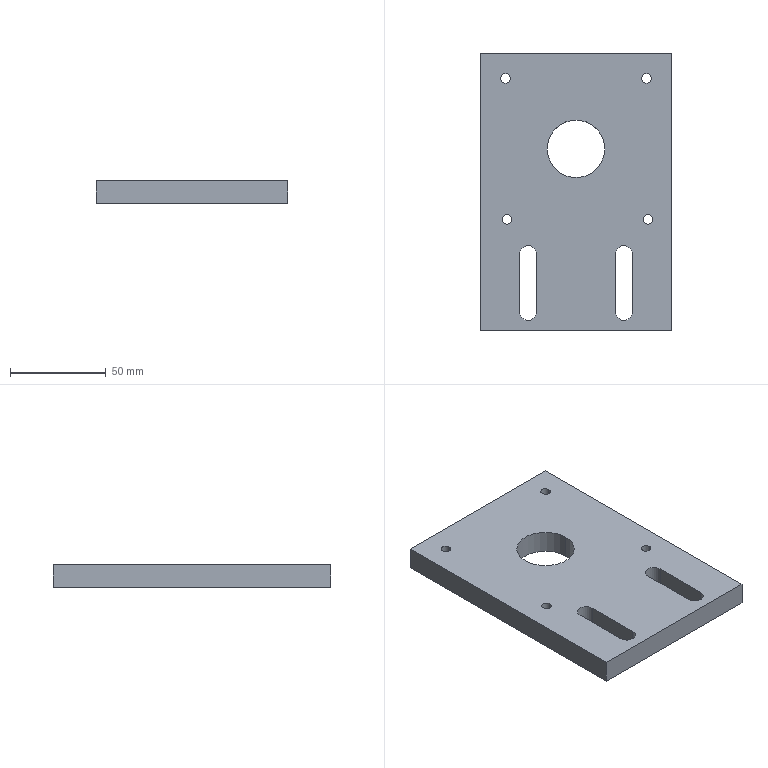Component | SolidWorks | MotorMount-2 | 1 solid | 24 faces | box 100 x 145 x 12 mm | volume 156568 mm3 | cylinder 14 | plane 10 | commonest cylinder face diameters 5 x8 9 x4 30 x2
build123d program:
from build123d import *

# Parameters (mm, degrees)
SKETCH1_W             = 100
SKETCH1_H             = 145
SKETCH1_R             = 15
EXTRUDE1_DEPTH        = 12
M6_TAPPED_HOLE1_D     = 5
M6_TAPPED_HOLE1_DEPTH = 17
M6_TAPPED_HOLE1_TIP   = 1.502


with BuildPart() as part:
    # Sketch1 → Extrude1 (new body)
    with BuildSketch(Plane.XY):
        with Locations((25.043, -0.7753)):
            Rectangle(SKETCH1_W, SKETCH1_H)
        with Locations((25.043, 21.725)):
            Circle(SKETCH1_R, mode=Mode.SUBTRACT)
        with BuildLine():
            Line((45.543, -33.275), (45.543, -63.275))
            ThreePointArc((45.543, -63.275), (50.043, -67.775), (54.543, -63.275))
            Line((54.543, -63.275), (54.543, -33.275))
            ThreePointArc((54.543, -33.275), (50.043, -28.775), (45.543, -33.275))
        make_face(mode=Mode.SUBTRACT)
        with BuildLine():
            Line((-4.457, -33.275), (-4.457, -63.275))
            ThreePointArc((-4.457, -63.275), (0.04302, -67.775), (4.543, -63.275))
            Line((4.543, -63.275), (4.543, -33.275))
            ThreePointArc((4.543, -33.275), (0.04302, -28.775), (-4.457, -33.275))
        make_face(mode=Mode.SUBTRACT)
    extrude(amount=EXTRUDE1_DEPTH)

    # M6 Tapped Hole1
    with Locations(Plane(origin=(0, 0, 0), x_dir=(-1, 0, 0), z_dir=(0, 0, -1))):
        with Locations((11.707, 58.475), (-61.793, 58.475), (-62.543, -15.021), (10.957, -15.025)):
            Hole(M6_TAPPED_HOLE1_D / 2, depth=M6_TAPPED_HOLE1_DEPTH)
            with Locations((0, 0, -(M6_TAPPED_HOLE1_DEPTH + M6_TAPPED_HOLE1_TIP / 2))):  # 118° drill point
                Cone(0, M6_TAPPED_HOLE1_D / 2, M6_TAPPED_HOLE1_TIP, mode=Mode.SUBTRACT)


solid = part.part

# Placed as in the assembly
solid = solid.moved(Location((-185.987, 672.259, 237.789), (0, 0, 0)))
STEP:
#1=COLOUR_RGB('',0.7922,0.8196,0.9333);
#2=FILL_AREA_STYLE_COLOUR('',#1);
#3=FILL_AREA_STYLE('',(#2));
#4=SURFACE_STYLE_FILL_AREA(#3);
#5=SURFACE_SIDE_STYLE('',(#4));
#6=SURFACE_STYLE_USAGE(.BOTH.,#5);
#7=PRESENTATION_STYLE_ASSIGNMENT((#6));
#8=CARTESIAN_POINT('',(-7.882,28.769,9.834));
#9=VERTEX_POINT('',#8);
#10=CARTESIAN_POINT('',(-7.685,28.769,9.834));
#11=VERTEX_POINT('',#10);
#12=CARTESIAN_POINT('',(-7.783,28.769,9.834));
#13=DIRECTION('',(0.,0.,1.));
#14=DIRECTION('',(1.,0.,0.));
#15=AXIS2_PLACEMENT_3D('',#12,#13,#14);
#16=CIRCLE('',#15,0.09843);
#17=EDGE_CURVE('',#9,#11,#16,.T.);
#18=ORIENTED_EDGE('',*,*,#17,.T.);
#19=CARTESIAN_POINT('',(-7.685,28.769,9.362));
#20=VERTEX_POINT('',#19);
#21=CARTESIAN_POINT('',(-7.685,28.769,9.362));
#22=DIRECTION('',(0.,0.,-1.));
#23=VECTOR('',#22,39.37);
#24=LINE('',#21,#23);
#25=EDGE_CURVE('',#11,#20,#24,.T.);
#26=ORIENTED_EDGE('',*,*,#25,.T.);
#27=CARTESIAN_POINT('',(-7.882,28.769,9.362));
#28=VERTEX_POINT('',#27);
#29=CARTESIAN_POINT('',(-7.783,28.769,9.362));
#30=DIRECTION('',(0.,0.,-1.));
#31=DIRECTION('',(-1.,0.,0.));
#32=AXIS2_PLACEMENT_3D('',#29,#30,#31);
#33=CIRCLE('',#32,0.09843);
#34=EDGE_CURVE('',#20,#28,#33,.T.);
#35=ORIENTED_EDGE('',*,*,#34,.T.);
#36=CARTESIAN_POINT('',(-7.882,28.769,9.362));
#37=DIRECTION('',(0.,0.,-1.));
#38=VECTOR('',#37,39.37);
#39=LINE('',#36,#38);
#40=EDGE_CURVE('',#9,#28,#39,.T.);
#41=ORIENTED_EDGE('',*,*,#40,.F.);
#42=EDGE_LOOP('',(#18,#26,#35,#41));
#43=FACE_OUTER_BOUND('',#42,.T.);
#44=CARTESIAN_POINT('',(-7.783,28.769,9.362));
#45=DIRECTION('',(0.,0.,-1.));
#46=DIRECTION('',(-1.,0.,0.));
#47=AXIS2_PLACEMENT_3D('',#44,#45,#46);
#48=CYLINDRICAL_SURFACE('',#47,0.09843);
#49=ADVANCED_FACE('',(#43),#48,.F.);
#50=CARTESIAN_POINT('',(-4.988,28.769,9.834));
#51=VERTEX_POINT('',#50);
#52=CARTESIAN_POINT('',(-4.791,28.769,9.834));
#53=VERTEX_POINT('',#52);
#54=CARTESIAN_POINT('',(-4.89,28.769,9.834));
#55=DIRECTION('',(0.,0.,1.));
#56=DIRECTION('',(1.,0.,0.));
#57=AXIS2_PLACEMENT_3D('',#54,#55,#56);
#58=CIRCLE('',#57,0.09843);
#59=EDGE_CURVE('',#51,#53,#58,.T.);
#60=ORIENTED_EDGE('',*,*,#59,.T.);
#61=CARTESIAN_POINT('',(-4.791,28.769,9.362));
#62=VERTEX_POINT('',#61);
#63=CARTESIAN_POINT('',(-4.791,28.769,9.362));
#64=DIRECTION('',(0.,0.,-1.));
#65=VECTOR('',#64,39.37);
#66=LINE('',#63,#65);
#67=EDGE_CURVE('',#53,#62,#66,.T.);
#68=ORIENTED_EDGE('',*,*,#67,.T.);
#69=CARTESIAN_POINT('',(-4.988,28.769,9.362));
#70=VERTEX_POINT('',#69);
#71=CARTESIAN_POINT('',(-4.89,28.769,9.362));
#72=DIRECTION('',(0.,0.,-1.));
#73=DIRECTION('',(-1.,0.,0.));
#74=AXIS2_PLACEMENT_3D('',#71,#72,#73);
#75=CIRCLE('',#74,0.09843);
#76=EDGE_CURVE('',#62,#70,#75,.T.);
#77=ORIENTED_EDGE('',*,*,#76,.T.);
#78=CARTESIAN_POINT('',(-4.988,28.769,9.362));
#79=DIRECTION('',(0.,0.,-1.));
#80=VECTOR('',#79,39.37);
#81=LINE('',#78,#80);
#82=EDGE_CURVE('',#51,#70,#81,.T.);
#83=ORIENTED_EDGE('',*,*,#82,.F.);
#84=EDGE_LOOP('',(#60,#68,#77,#83));
#85=FACE_OUTER_BOUND('',#84,.T.);
#86=CARTESIAN_POINT('',(-4.89,28.769,9.362));
#87=DIRECTION('',(0.,0.,-1.));
#88=DIRECTION('',(-1.,0.,0.));
#89=AXIS2_PLACEMENT_3D('',#86,#87,#88);
#90=CYLINDRICAL_SURFACE('',#89,0.09843);
#91=ADVANCED_FACE('',(#85),#90,.F.);
#92=CARTESIAN_POINT('',(-4.958,25.875,9.834));
#93=VERTEX_POINT('',#92);
#94=CARTESIAN_POINT('',(-4.762,25.875,9.834));
#95=VERTEX_POINT('',#94);
#96=CARTESIAN_POINT('',(-4.86,25.875,9.834));
#97=DIRECTION('',(0.,0.,1.));
#98=DIRECTION('',(1.,0.,0.));
#99=AXIS2_PLACEMENT_3D('',#96,#97,#98);
#100=CIRCLE('',#99,0.09843);
#101=EDGE_CURVE('',#93,#95,#100,.T.);
#102=ORIENTED_EDGE('',*,*,#101,.T.);
#103=CARTESIAN_POINT('',(-4.762,25.875,9.362));
#104=VERTEX_POINT('',#103);
#105=CARTESIAN_POINT('',(-4.762,25.875,9.362));
#106=DIRECTION('',(0.,0.,-1.));
#107=VECTOR('',#106,39.37);
#108=LINE('',#105,#107);
#109=EDGE_CURVE('',#95,#104,#108,.T.);
#110=ORIENTED_EDGE('',*,*,#109,.T.);
#111=CARTESIAN_POINT('',(-4.958,25.875,9.362));
#112=VERTEX_POINT('',#111);
#113=CARTESIAN_POINT('',(-4.86,25.875,9.362));
#114=DIRECTION('',(0.,0.,-1.));
#115=DIRECTION('',(-1.,0.,0.));
#116=AXIS2_PLACEMENT_3D('',#113,#114,#115);
#117=CIRCLE('',#116,0.09843);
#118=EDGE_CURVE('',#104,#112,#117,.T.);
#119=ORIENTED_EDGE('',*,*,#118,.T.);
#120=CARTESIAN_POINT('',(-4.958,25.875,9.362));
#121=DIRECTION('',(0.,0.,-1.));
#122=VECTOR('',#121,39.37);
#123=LINE('',#120,#122);
#124=EDGE_CURVE('',#93,#112,#123,.T.);
#125=ORIENTED_EDGE('',*,*,#124,.F.);
#126=EDGE_LOOP('',(#102,#110,#119,#125));
#127=FACE_OUTER_BOUND('',#126,.T.);
#128=CARTESIAN_POINT('',(-4.86,25.875,9.362));
#129=DIRECTION('',(0.,0.,-1.));
#130=DIRECTION('',(-1.,0.,0.));
#131=AXIS2_PLACEMENT_3D('',#128,#129,#130);
#132=CYLINDRICAL_SURFACE('',#131,0.09843);
#133=ADVANCED_FACE('',(#127),#132,.F.);
#134=CARTESIAN_POINT('',(-7.852,25.875,9.834));
#135=VERTEX_POINT('',#134);
#136=CARTESIAN_POINT('',(-7.655,25.875,9.834));
#137=VERTEX_POINT('',#136);
#138=CARTESIAN_POINT('',(-7.754,25.875,9.834));
#139=DIRECTION('',(0.,0.,1.));
#140=DIRECTION('',(1.,0.,0.));
#141=AXIS2_PLACEMENT_3D('',#138,#139,#140);
#142=CIRCLE('',#141,0.09843);
#143=EDGE_CURVE('',#135,#137,#142,.T.);
#144=ORIENTED_EDGE('',*,*,#143,.T.);
#145=CARTESIAN_POINT('',(-7.655,25.875,9.362));
#146=VERTEX_POINT('',#145);
#147=CARTESIAN_POINT('',(-7.655,25.875,9.362));
#148=DIRECTION('',(0.,0.,-1.));
#149=VECTOR('',#148,39.37);
#150=LINE('',#147,#149);
#151=EDGE_CURVE('',#137,#146,#150,.T.);
#152=ORIENTED_EDGE('',*,*,#151,.T.);
#153=CARTESIAN_POINT('',(-7.852,25.875,9.362));
#154=VERTEX_POINT('',#153);
#155=CARTESIAN_POINT('',(-7.754,25.875,9.362));
#156=DIRECTION('',(0.,0.,-1.));
#157=DIRECTION('',(-1.,0.,0.));
#158=AXIS2_PLACEMENT_3D('',#155,#156,#157);
#159=CIRCLE('',#158,0.09843);
#160=EDGE_CURVE('',#146,#154,#159,.T.);
#161=ORIENTED_EDGE('',*,*,#160,.T.);
#162=CARTESIAN_POINT('',(-7.852,25.875,9.362));
#163=DIRECTION('',(0.,0.,-1.));
#164=VECTOR('',#163,39.37);
#165=LINE('',#162,#164);
#166=EDGE_CURVE('',#135,#154,#165,.T.);
#167=ORIENTED_EDGE('',*,*,#166,.F.);
#168=EDGE_LOOP('',(#144,#152,#161,#167));
#169=FACE_OUTER_BOUND('',#168,.T.);
#170=CARTESIAN_POINT('',(-7.754,25.875,9.362));
#171=DIRECTION('',(0.,0.,-1.));
#172=DIRECTION('',(-1.,0.,0.));
#173=AXIS2_PLACEMENT_3D('',#170,#171,#172);
#174=CYLINDRICAL_SURFACE('',#173,0.09843);
#175=ADVANCED_FACE('',(#169),#174,.F.);
#176=CARTESIAN_POINT('',(-6.927,27.322,9.834));
#177=VERTEX_POINT('',#176);
#178=CARTESIAN_POINT('',(-5.746,27.322,9.834));
#179=VERTEX_POINT('',#178);
#180=CARTESIAN_POINT('',(-6.336,27.322,9.834));
#181=DIRECTION('',(0.,0.,1.));
#182=DIRECTION('',(1.,0.,0.));
#183=AXIS2_PLACEMENT_3D('',#180,#181,#182);
#184=CIRCLE('',#183,0.5906);
#185=EDGE_CURVE('',#177,#179,#184,.T.);
#186=ORIENTED_EDGE('',*,*,#185,.T.);
#187=CARTESIAN_POINT('',(-5.746,27.322,9.362));
#188=VERTEX_POINT('',#187);
#189=CARTESIAN_POINT('',(-5.746,27.322,9.834));
#190=DIRECTION('',(0.,0.,-1.));
#191=VECTOR('',#190,39.37);
#192=LINE('',#189,#191);
#193=EDGE_CURVE('',#179,#188,#192,.T.);
#194=ORIENTED_EDGE('',*,*,#193,.T.);
#195=CARTESIAN_POINT('',(-6.927,27.322,9.362));
#196=VERTEX_POINT('',#195);
#197=CARTESIAN_POINT('',(-6.336,27.322,9.362));
#198=DIRECTION('',(0.,0.,1.));
#199=DIRECTION('',(1.,0.,0.));
#200=AXIS2_PLACEMENT_3D('',#197,#198,#199);
#201=CIRCLE('',#200,0.5906);
#202=EDGE_CURVE('',#196,#188,#201,.T.);
#203=ORIENTED_EDGE('',*,*,#202,.F.);
#204=CARTESIAN_POINT('',(-6.927,27.322,9.834));
#205=DIRECTION('',(0.,0.,-1.));
#206=VECTOR('',#205,39.37);
#207=LINE('',#204,#206);
#208=EDGE_CURVE('',#177,#196,#207,.T.);
#209=ORIENTED_EDGE('',*,*,#208,.F.);
#210=EDGE_LOOP('',(#186,#194,#203,#209));
#211=FACE_OUTER_BOUND('',#210,.T.);
#212=CARTESIAN_POINT('',(-6.336,27.322,9.834));
#213=DIRECTION('',(0.,0.,-1.));
#214=DIRECTION('',(-1.,0.,0.));
#215=AXIS2_PLACEMENT_3D('',#212,#213,#214);
#216=CYLINDRICAL_SURFACE('',#215,0.5906);
#217=ADVANCED_FACE('',(#211),#216,.F.);
#218=ORIENTED_EDGE('',*,*,#17,.F.);
#219=CARTESIAN_POINT('',(-7.783,28.769,9.834));
#220=DIRECTION('',(0.,0.,1.));
#221=DIRECTION('',(1.,0.,0.));
#222=AXIS2_PLACEMENT_3D('',#219,#220,#221);
#223=CIRCLE('',#222,0.09843);
#224=EDGE_CURVE('',#11,#9,#223,.T.);
#225=ORIENTED_EDGE('',*,*,#224,.F.);
#226=EDGE_LOOP('',(#218,#225));
#227=FACE_BOUND('',#226,.T.);
#228=ORIENTED_EDGE('',*,*,#59,.F.);
#229=CARTESIAN_POINT('',(-4.89,28.769,9.834));
#230=DIRECTION('',(0.,0.,1.));
#231=DIRECTION('',(1.,0.,0.));
#232=AXIS2_PLACEMENT_3D('',#229,#230,#231);
#233=CIRCLE('',#232,0.09843);
#234=EDGE_CURVE('',#53,#51,#233,.T.);
#235=ORIENTED_EDGE('',*,*,#234,.F.);
#236=EDGE_LOOP('',(#228,#235));
#237=FACE_BOUND('',#236,.T.);
#238=ORIENTED_EDGE('',*,*,#101,.F.);
#239=CARTESIAN_POINT('',(-4.86,25.875,9.834));
#240=DIRECTION('',(0.,0.,1.));
#241=DIRECTION('',(1.,0.,0.));
#242=AXIS2_PLACEMENT_3D('',#239,#240,#241);
#243=CIRCLE('',#242,0.09843);
#244=EDGE_CURVE('',#95,#93,#243,.T.);
#245=ORIENTED_EDGE('',*,*,#244,.F.);
#246=EDGE_LOOP('',(#238,#245));
#247=FACE_BOUND('',#246,.T.);
#248=ORIENTED_EDGE('',*,*,#143,.F.);
#249=CARTESIAN_POINT('',(-7.754,25.875,9.834));
#250=DIRECTION('',(0.,0.,1.));
#251=DIRECTION('',(1.,0.,0.));
#252=AXIS2_PLACEMENT_3D('',#249,#250,#251);
#253=CIRCLE('',#252,0.09843);
#254=EDGE_CURVE('',#137,#135,#253,.T.);
#255=ORIENTED_EDGE('',*,*,#254,.F.);
#256=EDGE_LOOP('',(#248,#255));
#257=FACE_BOUND('',#256,.T.);
#258=CARTESIAN_POINT('',(-8.305,29.291,9.834));
#259=VERTEX_POINT('',#258);
#260=CARTESIAN_POINT('',(-8.305,23.582,9.834));
#261=VERTEX_POINT('',#260);
#262=CARTESIAN_POINT('',(-8.305,29.291,9.834));
#263=DIRECTION('',(0.,-1.,0.));
#264=VECTOR('',#263,39.37);
#265=LINE('',#262,#264);
#266=EDGE_CURVE('',#259,#261,#265,.T.);
#267=ORIENTED_EDGE('',*,*,#266,.T.);
#268=CARTESIAN_POINT('',(-4.368,23.582,9.834));
#269=VERTEX_POINT('',#268);
#270=CARTESIAN_POINT('',(-8.305,23.582,9.834));
#271=DIRECTION('',(1.,0.,0.));
#272=VECTOR('',#271,39.37);
#273=LINE('',#270,#272);
#274=EDGE_CURVE('',#261,#269,#273,.T.);
#275=ORIENTED_EDGE('',*,*,#274,.T.);
#276=CARTESIAN_POINT('',(-4.368,29.291,9.834));
#277=VERTEX_POINT('',#276);
#278=CARTESIAN_POINT('',(-4.368,29.291,9.834));
#279=DIRECTION('',(-0.,1.,0.));
#280=VECTOR('',#279,39.37);
#281=LINE('',#278,#280);
#282=EDGE_CURVE('',#269,#277,#281,.T.);
#283=ORIENTED_EDGE('',*,*,#282,.T.);
#284=CARTESIAN_POINT('',(-8.305,29.291,9.834));
#285=DIRECTION('',(-1.,0.,0.));
#286=VECTOR('',#285,39.37);
#287=LINE('',#284,#286);
#288=EDGE_CURVE('',#277,#259,#287,.T.);
#289=ORIENTED_EDGE('',*,*,#288,.T.);
#290=EDGE_LOOP('',(#267,#275,#283,#289));
#291=FACE_OUTER_BOUND('',#290,.T.);
#292=ORIENTED_EDGE('',*,*,#185,.F.);
#293=CARTESIAN_POINT('',(-6.336,27.322,9.834));
#294=DIRECTION('',(0.,0.,1.));
#295=DIRECTION('',(1.,0.,0.));
#296=AXIS2_PLACEMENT_3D('',#293,#294,#295);
#297=CIRCLE('',#296,0.5906);
#298=EDGE_CURVE('',#179,#177,#297,.T.);
#299=ORIENTED_EDGE('',*,*,#298,.F.);
#300=EDGE_LOOP('',(#292,#299));
#301=FACE_BOUND('',#300,.T.);
#302=CARTESIAN_POINT('',(-7.498,25.157,9.834));
#303=VERTEX_POINT('',#302);
#304=CARTESIAN_POINT('',(-7.498,23.976,9.834));
#305=VERTEX_POINT('',#304);
#306=CARTESIAN_POINT('',(-7.498,25.157,9.834));
#307=DIRECTION('',(0.,-1.,0.));
#308=VECTOR('',#307,39.37);
#309=LINE('',#306,#308);
#310=EDGE_CURVE('',#303,#305,#309,.T.);
#311=ORIENTED_EDGE('',*,*,#310,.F.);
#312=CARTESIAN_POINT('',(-7.143,25.157,9.834));
#313=VERTEX_POINT('',#312);
#314=CARTESIAN_POINT('',(-7.321,25.157,9.834));
#315=DIRECTION('',(0.,0.,1.));
#316=DIRECTION('',(1.,0.,0.));
#317=AXIS2_PLACEMENT_3D('',#314,#315,#316);
#318=CIRCLE('',#317,0.1772);
#319=EDGE_CURVE('',#313,#303,#318,.T.);
#320=ORIENTED_EDGE('',*,*,#319,.F.);
#321=CARTESIAN_POINT('',(-7.143,23.976,9.834));
#322=VERTEX_POINT('',#321);
#323=CARTESIAN_POINT('',(-7.143,25.157,9.834));
#324=DIRECTION('',(-0.,1.,0.));
#325=VECTOR('',#324,39.37);
#326=LINE('',#323,#325);
#327=EDGE_CURVE('',#322,#313,#326,.T.);
#328=ORIENTED_EDGE('',*,*,#327,.F.);
#329=CARTESIAN_POINT('',(-7.321,23.976,9.834));
#330=DIRECTION('',(0.,0.,1.));
#331=DIRECTION('',(1.,0.,0.));
#332=AXIS2_PLACEMENT_3D('',#329,#330,#331);
#333=CIRCLE('',#332,0.1772);
#334=EDGE_CURVE('',#305,#322,#333,.T.);
#335=ORIENTED_EDGE('',*,*,#334,.F.);
#336=EDGE_LOOP('',(#311,#320,#328,#335));
#337=FACE_BOUND('',#336,.T.);
#338=CARTESIAN_POINT('',(-5.175,23.976,9.834));
#339=VERTEX_POINT('',#338);
#340=CARTESIAN_POINT('',(-5.175,25.157,9.834));
#341=VERTEX_POINT('',#340);
#342=CARTESIAN_POINT('',(-5.175,25.157,9.834));
#343=DIRECTION('',(-0.,1.,0.));
#344=VECTOR('',#343,39.37);
#345=LINE('',#342,#344);
#346=EDGE_CURVE('',#339,#341,#345,.T.);
#347=ORIENTED_EDGE('',*,*,#346,.F.);
#348=CARTESIAN_POINT('',(-5.529,23.976,9.834));
#349=VERTEX_POINT('',#348);
#350=CARTESIAN_POINT('',(-5.352,23.976,9.834));
#351=DIRECTION('',(0.,0.,1.));
#352=DIRECTION('',(-1.,0.,0.));
#353=AXIS2_PLACEMENT_3D('',#350,#351,#352);
#354=CIRCLE('',#353,0.1772);
#355=EDGE_CURVE('',#349,#339,#354,.T.);
#356=ORIENTED_EDGE('',*,*,#355,.F.);
#357=CARTESIAN_POINT('',(-5.529,25.157,9.834));
#358=VERTEX_POINT('',#357);
#359=CARTESIAN_POINT('',(-5.529,25.157,9.834));
#360=DIRECTION('',(0.,-1.,0.));
#361=VECTOR('',#360,39.37);
#362=LINE('',#359,#361);
#363=EDGE_CURVE('',#358,#349,#362,.T.);
#364=ORIENTED_EDGE('',*,*,#363,.F.);
#365=CARTESIAN_POINT('',(-5.352,25.157,9.834));
#366=DIRECTION('',(0.,0.,1.));
#367=DIRECTION('',(-1.,0.,0.));
#368=AXIS2_PLACEMENT_3D('',#365,#366,#367);
#369=CIRCLE('',#368,0.1772);
#370=EDGE_CURVE('',#341,#358,#369,.T.);
#371=ORIENTED_EDGE('',*,*,#370,.F.);
#372=EDGE_LOOP('',(#347,#356,#364,#371));
#373=FACE_BOUND('',#372,.T.);
#374=CARTESIAN_POINT('',(-8.305,23.582,9.834));
#375=DIRECTION('',(0.,0.,1.));
#376=DIRECTION('',(1.,0.,0.));
#377=AXIS2_PLACEMENT_3D('',#374,#375,#376);
#378=PLANE('',#377);
#379=ADVANCED_FACE('',(#227,#237,#247,#257,#291,#301,#337,#373),#378,.T.);
#380=CARTESIAN_POINT('',(-7.783,28.769,9.362));
#381=DIRECTION('',(0.,0.,-1.));
#382=DIRECTION('',(-1.,0.,0.));
#383=AXIS2_PLACEMENT_3D('',#380,#381,#382);
#384=CIRCLE('',#383,0.09843);
#385=EDGE_CURVE('',#28,#20,#384,.T.);
#386=ORIENTED_EDGE('',*,*,#385,.F.);
#387=ORIENTED_EDGE('',*,*,#34,.F.);
#388=EDGE_LOOP('',(#386,#387));
#389=FACE_BOUND('',#388,.T.);
#390=CARTESIAN_POINT('',(-4.89,28.769,9.362));
#391=DIRECTION('',(0.,0.,-1.));
#392=DIRECTION('',(-1.,0.,0.));
#393=AXIS2_PLACEMENT_3D('',#390,#391,#392);
#394=CIRCLE('',#393,0.09843);
#395=EDGE_CURVE('',#70,#62,#394,.T.);
#396=ORIENTED_EDGE('',*,*,#395,.F.);
#397=ORIENTED_EDGE('',*,*,#76,.F.);
#398=EDGE_LOOP('',(#396,#397));
#399=FACE_BOUND('',#398,.T.);
#400=CARTESIAN_POINT('',(-4.86,25.875,9.362));
#401=DIRECTION('',(0.,0.,-1.));
#402=DIRECTION('',(-1.,0.,0.));
#403=AXIS2_PLACEMENT_3D('',#400,#401,#402);
#404=CIRCLE('',#403,0.09843);
#405=EDGE_CURVE('',#112,#104,#404,.T.);
#406=ORIENTED_EDGE('',*,*,#405,.F.);
#407=ORIENTED_EDGE('',*,*,#118,.F.);
#408=EDGE_LOOP('',(#406,#407));
#409=FACE_BOUND('',#408,.T.);
#410=CARTESIAN_POINT('',(-7.754,25.875,9.362));
#411=DIRECTION('',(0.,0.,-1.));
#412=DIRECTION('',(-1.,0.,0.));
#413=AXIS2_PLACEMENT_3D('',#410,#411,#412);
#414=CIRCLE('',#413,0.09843);
#415=EDGE_CURVE('',#154,#146,#414,.T.);
#416=ORIENTED_EDGE('',*,*,#415,.F.);
#417=ORIENTED_EDGE('',*,*,#160,.F.);
#418=EDGE_LOOP('',(#416,#417));
#419=FACE_BOUND('',#418,.T.);
#420=CARTESIAN_POINT('',(-7.143,25.157,9.362));
#421=VERTEX_POINT('',#420);
#422=CARTESIAN_POINT('',(-7.498,25.157,9.362));
#423=VERTEX_POINT('',#422);
#424=CARTESIAN_POINT('',(-7.321,25.157,9.362));
#425=DIRECTION('',(0.,0.,1.));
#426=DIRECTION('',(1.,0.,0.));
#427=AXIS2_PLACEMENT_3D('',#424,#425,#426);
#428=CIRCLE('',#427,0.1772);
#429=EDGE_CURVE('',#421,#423,#428,.T.);
#430=ORIENTED_EDGE('',*,*,#429,.T.);
#431=CARTESIAN_POINT('',(-7.498,23.976,9.362));
#432=VERTEX_POINT('',#431);
#433=CARTESIAN_POINT('',(-7.498,25.157,9.362));
#434=DIRECTION('',(0.,-1.,0.));
#435=VECTOR('',#434,39.37);
#436=LINE('',#433,#435);
#437=EDGE_CURVE('',#423,#432,#436,.T.);
#438=ORIENTED_EDGE('',*,*,#437,.T.);
#439=CARTESIAN_POINT('',(-7.143,23.976,9.362));
#440=VERTEX_POINT('',#439);
#441=CARTESIAN_POINT('',(-7.321,23.976,9.362));
#442=DIRECTION('',(0.,0.,1.));
#443=DIRECTION('',(1.,0.,0.));
#444=AXIS2_PLACEMENT_3D('',#441,#442,#443);
#445=CIRCLE('',#444,0.1772);
#446=EDGE_CURVE('',#432,#440,#445,.T.);
#447=ORIENTED_EDGE('',*,*,#446,.T.);
#448=CARTESIAN_POINT('',(-7.143,25.157,9.362));
#449=DIRECTION('',(-0.,1.,0.));
#450=VECTOR('',#449,39.37);
#451=LINE('',#448,#450);
#452=EDGE_CURVE('',#440,#421,#451,.T.);
#453=ORIENTED_EDGE('',*,*,#452,.T.);
#454=EDGE_LOOP('',(#430,#438,#447,#453));
#455=FACE_BOUND('',#454,.T.);
#456=CARTESIAN_POINT('',(-8.305,29.291,9.362));
#457=VERTEX_POINT('',#456);
#458=CARTESIAN_POINT('',(-8.305,23.582,9.362));
#459=VERTEX_POINT('',#458);
#460=CARTESIAN_POINT('',(-8.305,29.291,9.362));
#461=DIRECTION('',(0.,-1.,0.));
#462=VECTOR('',#461,39.37);
#463=LINE('',#460,#462);
#464=EDGE_CURVE('',#457,#459,#463,.T.);
#465=ORIENTED_EDGE('',*,*,#464,.F.);
#466=CARTESIAN_POINT('',(-4.368,29.291,9.362));
#467=VERTEX_POINT('',#466);
#468=CARTESIAN_POINT('',(-8.305,29.291,9.362));
#469=DIRECTION('',(-1.,0.,0.));
#470=VECTOR('',#469,39.37);
#471=LINE('',#468,#470);
#472=EDGE_CURVE('',#467,#457,#471,.T.);
#473=ORIENTED_EDGE('',*,*,#472,.F.);
#474=CARTESIAN_POINT('',(-4.368,23.582,9.362));
#475=VERTEX_POINT('',#474);
#476=CARTESIAN_POINT('',(-4.368,29.291,9.362));
#477=DIRECTION('',(-0.,1.,0.));
#478=VECTOR('',#477,39.37);
#479=LINE('',#476,#478);
#480=EDGE_CURVE('',#475,#467,#479,.T.);
#481=ORIENTED_EDGE('',*,*,#480,.F.);
#482=CARTESIAN_POINT('',(-8.305,23.582,9.362));
#483=DIRECTION('',(1.,0.,0.));
#484=VECTOR('',#483,39.37);
#485=LINE('',#482,#484);
#486=EDGE_CURVE('',#459,#475,#485,.T.);
#487=ORIENTED_EDGE('',*,*,#486,.F.);
#488=EDGE_LOOP('',(#465,#473,#481,#487));
#489=FACE_OUTER_BOUND('',#488,.T.);
#490=ORIENTED_EDGE('',*,*,#202,.T.);
#491=CARTESIAN_POINT('',(-6.336,27.322,9.362));
#492=DIRECTION('',(0.,0.,1.));
#493=DIRECTION('',(1.,0.,0.));
#494=AXIS2_PLACEMENT_3D('',#491,#492,#493);
#495=CIRCLE('',#494,0.5906);
#496=EDGE_CURVE('',#188,#196,#495,.T.);
#497=ORIENTED_EDGE('',*,*,#496,.T.);
#498=EDGE_LOOP('',(#490,#497));
#499=FACE_BOUND('',#498,.T.);
#500=CARTESIAN_POINT('',(-5.529,23.976,9.362));
#501=VERTEX_POINT('',#500);
#502=CARTESIAN_POINT('',(-5.175,23.976,9.362));
#503=VERTEX_POINT('',#502);
#504=CARTESIAN_POINT('',(-5.352,23.976,9.362));
#505=DIRECTION('',(0.,0.,1.));
#506=DIRECTION('',(-1.,0.,0.));
#507=AXIS2_PLACEMENT_3D('',#504,#505,#506);
#508=CIRCLE('',#507,0.1772);
#509=EDGE_CURVE('',#501,#503,#508,.T.);
#510=ORIENTED_EDGE('',*,*,#509,.T.);
#511=CARTESIAN_POINT('',(-5.175,25.157,9.362));
#512=VERTEX_POINT('',#511);
#513=CARTESIAN_POINT('',(-5.175,25.157,9.362));
#514=DIRECTION('',(-0.,1.,0.));
#515=VECTOR('',#514,39.37);
#516=LINE('',#513,#515);
#517=EDGE_CURVE('',#503,#512,#516,.T.);
#518=ORIENTED_EDGE('',*,*,#517,.T.);
#519=CARTESIAN_POINT('',(-5.529,25.157,9.362));
#520=VERTEX_POINT('',#519);
#521=CARTESIAN_POINT('',(-5.352,25.157,9.362));
#522=DIRECTION('',(0.,0.,1.));
#523=DIRECTION('',(-1.,0.,0.));
#524=AXIS2_PLACEMENT_3D('',#521,#522,#523);
#525=CIRCLE('',#524,0.1772);
#526=EDGE_CURVE('',#512,#520,#525,.T.);
#527=ORIENTED_EDGE('',*,*,#526,.T.);
#528=CARTESIAN_POINT('',(-5.529,25.157,9.362));
#529=DIRECTION('',(0.,-1.,0.));
#530=VECTOR('',#529,39.37);
#531=LINE('',#528,#530);
#532=EDGE_CURVE('',#520,#501,#531,.T.);
#533=ORIENTED_EDGE('',*,*,#532,.T.);
#534=EDGE_LOOP('',(#510,#518,#527,#533));
#535=FACE_BOUND('',#534,.T.);
#536=CARTESIAN_POINT('',(-8.305,23.582,9.362));
#537=DIRECTION('',(0.,0.,1.));
#538=DIRECTION('',(1.,0.,0.));
#539=AXIS2_PLACEMENT_3D('',#536,#537,#538);
#540=PLANE('',#539);
#541=ADVANCED_FACE('',(#389,#399,#409,#419,#455,#489,#499,#535),#540,.F.);
#542=ORIENTED_EDGE('',*,*,#464,.T.);
#543=CARTESIAN_POINT('',(-8.305,23.582,9.834));
#544=DIRECTION('',(0.,0.,-1.));
#545=VECTOR('',#544,39.37);
#546=LINE('',#543,#545);
#547=EDGE_CURVE('',#261,#459,#546,.T.);
#548=ORIENTED_EDGE('',*,*,#547,.F.);
#549=ORIENTED_EDGE('',*,*,#266,.F.);
#550=CARTESIAN_POINT('',(-8.305,29.291,9.834));
#551=DIRECTION('',(0.,0.,-1.));
#552=VECTOR('',#551,39.37);
#553=LINE('',#550,#552);
#554=EDGE_CURVE('',#259,#457,#553,.T.);
#555=ORIENTED_EDGE('',*,*,#554,.T.);
#556=EDGE_LOOP('',(#542,#548,#549,#555));
#557=FACE_OUTER_BOUND('',#556,.T.);
#558=CARTESIAN_POINT('',(-8.305,29.291,9.834));
#559=DIRECTION('',(1.,0.,0.));
#560=DIRECTION('',(-0.,1.,0.));
#561=AXIS2_PLACEMENT_3D('',#558,#559,#560);
#562=PLANE('',#561);
#563=ADVANCED_FACE('',(#557),#562,.F.);
#564=ORIENTED_EDGE('',*,*,#486,.T.);
#565=CARTESIAN_POINT('',(-4.368,23.582,9.834));
#566=DIRECTION('',(0.,0.,-1.));
#567=VECTOR('',#566,39.37);
#568=LINE('',#565,#567);
#569=EDGE_CURVE('',#269,#475,#568,.T.);
#570=ORIENTED_EDGE('',*,*,#569,.F.);
#571=ORIENTED_EDGE('',*,*,#274,.F.);
#572=ORIENTED_EDGE('',*,*,#547,.T.);
#573=EDGE_LOOP('',(#564,#570,#571,#572));
#574=FACE_OUTER_BOUND('',#573,.T.);
#575=CARTESIAN_POINT('',(-8.305,23.582,9.834));
#576=DIRECTION('',(-0.,1.,0.));
#577=DIRECTION('',(-1.,-0.,0.));
#578=AXIS2_PLACEMENT_3D('',#575,#576,#577);
#579=PLANE('',#578);
#580=ADVANCED_FACE('',(#574),#579,.F.);
#581=ORIENTED_EDGE('',*,*,#480,.T.);
#582=CARTESIAN_POINT('',(-4.368,29.291,9.834));
#583=DIRECTION('',(0.,0.,-1.));
#584=VECTOR('',#583,39.37);
#585=LINE('',#582,#584);
#586=EDGE_CURVE('',#277,#467,#585,.T.);
#587=ORIENTED_EDGE('',*,*,#586,.F.);
#588=ORIENTED_EDGE('',*,*,#282,.F.);
#589=ORIENTED_EDGE('',*,*,#569,.T.);
#590=EDGE_LOOP('',(#581,#587,#588,#589));
#591=FACE_OUTER_BOUND('',#590,.T.);
#592=CARTESIAN_POINT('',(-4.368,29.291,9.834));
#593=DIRECTION('',(-1.,-0.,0.));
#594=DIRECTION('',(0.,-1.,0.));
#595=AXIS2_PLACEMENT_3D('',#592,#593,#594);
#596=PLANE('',#595);
#597=ADVANCED_FACE('',(#591),#596,.F.);
#598=ORIENTED_EDGE('',*,*,#472,.T.);
#599=ORIENTED_EDGE('',*,*,#554,.F.);
#600=ORIENTED_EDGE('',*,*,#288,.F.);
#601=ORIENTED_EDGE('',*,*,#586,.T.);
#602=EDGE_LOOP('',(#598,#599,#600,#601));
#603=FACE_OUTER_BOUND('',#602,.T.);
#604=CARTESIAN_POINT('',(-8.305,29.291,9.834));
#605=DIRECTION('',(0.,-1.,0.));
#606=DIRECTION('',(0.,0.,-1.));
#607=AXIS2_PLACEMENT_3D('',#604,#605,#606);
#608=PLANE('',#607);
#609=ADVANCED_FACE('',(#603),#608,.F.);
#610=ORIENTED_EDGE('',*,*,#193,.F.);
#611=ORIENTED_EDGE('',*,*,#298,.T.);
#612=ORIENTED_EDGE('',*,*,#208,.T.);
#613=ORIENTED_EDGE('',*,*,#496,.F.);
#614=EDGE_LOOP('',(#610,#611,#612,#613));
#615=FACE_OUTER_BOUND('',#614,.T.);
#616=CARTESIAN_POINT('',(-6.336,27.322,9.834));
#617=DIRECTION('',(0.,0.,-1.));
#618=DIRECTION('',(-1.,0.,0.));
#619=AXIS2_PLACEMENT_3D('',#616,#617,#618);
#620=CYLINDRICAL_SURFACE('',#619,0.5906);
#621=ADVANCED_FACE('',(#615),#620,.F.);
#622=ORIENTED_EDGE('',*,*,#429,.F.);
#623=CARTESIAN_POINT('',(-7.143,25.157,9.834));
#624=DIRECTION('',(0.,0.,-1.));
#625=VECTOR('',#624,39.37);
#626=LINE('',#623,#625);
#627=EDGE_CURVE('',#313,#421,#626,.T.);
#628=ORIENTED_EDGE('',*,*,#627,.F.);
#629=ORIENTED_EDGE('',*,*,#319,.T.);
#630=CARTESIAN_POINT('',(-7.498,25.157,9.834));
#631=DIRECTION('',(0.,0.,-1.));
#632=VECTOR('',#631,39.37);
#633=LINE('',#630,#632);
#634=EDGE_CURVE('',#303,#423,#633,.T.);
#635=ORIENTED_EDGE('',*,*,#634,.T.);
#636=EDGE_LOOP('',(#622,#628,#629,#635));
#637=FACE_OUTER_BOUND('',#636,.T.);
#638=CARTESIAN_POINT('',(-7.321,25.157,9.834));
#639=DIRECTION('',(0.,0.,-1.));
#640=DIRECTION('',(-1.,0.,0.));
#641=AXIS2_PLACEMENT_3D('',#638,#639,#640);
#642=CYLINDRICAL_SURFACE('',#641,0.1772);
#643=ADVANCED_FACE('',(#637),#642,.F.);
#644=ORIENTED_EDGE('',*,*,#437,.F.);
#645=ORIENTED_EDGE('',*,*,#634,.F.);
#646=ORIENTED_EDGE('',*,*,#310,.T.);
#647=CARTESIAN_POINT('',(-7.498,23.976,9.834));
#648=DIRECTION('',(0.,0.,-1.));
#649=VECTOR('',#648,39.37);
#650=LINE('',#647,#649);
#651=EDGE_CURVE('',#305,#432,#650,.T.);
#652=ORIENTED_EDGE('',*,*,#651,.T.);
#653=EDGE_LOOP('',(#644,#645,#646,#652));
#654=FACE_OUTER_BOUND('',#653,.T.);
#655=CARTESIAN_POINT('',(-7.498,25.157,9.834));
#656=DIRECTION('',(1.,0.,0.));
#657=DIRECTION('',(-0.,1.,0.));
#658=AXIS2_PLACEMENT_3D('',#655,#656,#657);
#659=PLANE('',#658);
#660=ADVANCED_FACE('',(#654),#659,.T.);
#661=ORIENTED_EDGE('',*,*,#446,.F.);
#662=ORIENTED_EDGE('',*,*,#651,.F.);
#663=ORIENTED_EDGE('',*,*,#334,.T.);
#664=CARTESIAN_POINT('',(-7.143,23.976,9.834));
#665=DIRECTION('',(0.,0.,-1.));
#666=VECTOR('',#665,39.37);
#667=LINE('',#664,#666);
#668=EDGE_CURVE('',#322,#440,#667,.T.);
#669=ORIENTED_EDGE('',*,*,#668,.T.);
#670=EDGE_LOOP('',(#661,#662,#663,#669));
#671=FACE_OUTER_BOUND('',#670,.T.);
#672=CARTESIAN_POINT('',(-7.321,23.976,9.834));
#673=DIRECTION('',(0.,0.,-1.));
#674=DIRECTION('',(-1.,0.,0.));
#675=AXIS2_PLACEMENT_3D('',#672,#673,#674);
#676=CYLINDRICAL_SURFACE('',#675,0.1772);
#677=ADVANCED_FACE('',(#671),#676,.F.);
#678=ORIENTED_EDGE('',*,*,#452,.F.);
#679=ORIENTED_EDGE('',*,*,#668,.F.);
#680=ORIENTED_EDGE('',*,*,#327,.T.);
#681=ORIENTED_EDGE('',*,*,#627,.T.);
#682=EDGE_LOOP('',(#678,#679,#680,#681));
#683=FACE_OUTER_BOUND('',#682,.T.);
#684=CARTESIAN_POINT('',(-7.143,25.157,9.834));
#685=DIRECTION('',(-1.,-0.,0.));
#686=DIRECTION('',(0.,-1.,0.));
#687=AXIS2_PLACEMENT_3D('',#684,#685,#686);
#688=PLANE('',#687);
#689=ADVANCED_FACE('',(#683),#688,.T.);
#690=ORIENTED_EDGE('',*,*,#509,.F.);
#691=CARTESIAN_POINT('',(-5.529,23.976,9.834));
#692=DIRECTION('',(0.,0.,-1.));
#693=VECTOR('',#692,39.37);
#694=LINE('',#691,#693);
#695=EDGE_CURVE('',#349,#501,#694,.T.);
#696=ORIENTED_EDGE('',*,*,#695,.F.);
#697=ORIENTED_EDGE('',*,*,#355,.T.);
#698=CARTESIAN_POINT('',(-5.175,23.976,9.834));
#699=DIRECTION('',(0.,0.,-1.));
#700=VECTOR('',#699,39.37);
#701=LINE('',#698,#700);
#702=EDGE_CURVE('',#339,#503,#701,.T.);
#703=ORIENTED_EDGE('',*,*,#702,.T.);
#704=EDGE_LOOP('',(#690,#696,#697,#703));
#705=FACE_OUTER_BOUND('',#704,.T.);
#706=CARTESIAN_POINT('',(-5.352,23.976,9.834));
#707=DIRECTION('',(0.,0.,-1.));
#708=DIRECTION('',(-1.,0.,0.));
#709=AXIS2_PLACEMENT_3D('',#706,#707,#708);
#710=CYLINDRICAL_SURFACE('',#709,0.1772);
#711=ADVANCED_FACE('',(#705),#710,.F.);
#712=ORIENTED_EDGE('',*,*,#517,.F.);
#713=ORIENTED_EDGE('',*,*,#702,.F.);
#714=ORIENTED_EDGE('',*,*,#346,.T.);
#715=CARTESIAN_POINT('',(-5.175,25.157,9.834));
#716=DIRECTION('',(0.,0.,-1.));
#717=VECTOR('',#716,39.37);
#718=LINE('',#715,#717);
#719=EDGE_CURVE('',#341,#512,#718,.T.);
#720=ORIENTED_EDGE('',*,*,#719,.T.);
#721=EDGE_LOOP('',(#712,#713,#714,#720));
#722=FACE_OUTER_BOUND('',#721,.T.);
#723=CARTESIAN_POINT('',(-5.175,25.157,9.834));
#724=DIRECTION('',(-1.,-0.,0.));
#725=DIRECTION('',(0.,-1.,0.));
#726=AXIS2_PLACEMENT_3D('',#723,#724,#725);
#727=PLANE('',#726);
#728=ADVANCED_FACE('',(#722),#727,.T.);
#729=ORIENTED_EDGE('',*,*,#526,.F.);
#730=ORIENTED_EDGE('',*,*,#719,.F.);
#731=ORIENTED_EDGE('',*,*,#370,.T.);
#732=CARTESIAN_POINT('',(-5.529,25.157,9.834));
#733=DIRECTION('',(0.,0.,-1.));
#734=VECTOR('',#733,39.37);
#735=LINE('',#732,#734);
#736=EDGE_CURVE('',#358,#520,#735,.T.);
#737=ORIENTED_EDGE('',*,*,#736,.T.);
#738=EDGE_LOOP('',(#729,#730,#731,#737));
#739=FACE_OUTER_BOUND('',#738,.T.);
#740=CARTESIAN_POINT('',(-5.352,25.157,9.834));
#741=DIRECTION('',(0.,0.,-1.));
#742=DIRECTION('',(-1.,0.,0.));
#743=AXIS2_PLACEMENT_3D('',#740,#741,#742);
#744=CYLINDRICAL_SURFACE('',#743,0.1772);
#745=ADVANCED_FACE('',(#739),#744,.F.);
#746=ORIENTED_EDGE('',*,*,#532,.F.);
#747=ORIENTED_EDGE('',*,*,#736,.F.);
#748=ORIENTED_EDGE('',*,*,#363,.T.);
#749=ORIENTED_EDGE('',*,*,#695,.T.);
#750=EDGE_LOOP('',(#746,#747,#748,#749));
#751=FACE_OUTER_BOUND('',#750,.T.);
#752=CARTESIAN_POINT('',(-5.529,25.157,9.834));
#753=DIRECTION('',(1.,0.,0.));
#754=DIRECTION('',(-0.,1.,0.));
#755=AXIS2_PLACEMENT_3D('',#752,#753,#754);
#756=PLANE('',#755);
#757=ADVANCED_FACE('',(#751),#756,.T.);
#758=ORIENTED_EDGE('',*,*,#151,.F.);
#759=ORIENTED_EDGE('',*,*,#254,.T.);
#760=ORIENTED_EDGE('',*,*,#166,.T.);
#761=ORIENTED_EDGE('',*,*,#415,.T.);
#762=EDGE_LOOP('',(#758,#759,#760,#761));
#763=FACE_OUTER_BOUND('',#762,.T.);
#764=CARTESIAN_POINT('',(-7.754,25.875,9.362));
#765=DIRECTION('',(0.,0.,-1.));
#766=DIRECTION('',(-1.,0.,0.));
#767=AXIS2_PLACEMENT_3D('',#764,#765,#766);
#768=CYLINDRICAL_SURFACE('',#767,0.09843);
#769=ADVANCED_FACE('',(#763),#768,.F.);
#770=ORIENTED_EDGE('',*,*,#109,.F.);
#771=ORIENTED_EDGE('',*,*,#244,.T.);
#772=ORIENTED_EDGE('',*,*,#124,.T.);
#773=ORIENTED_EDGE('',*,*,#405,.T.);
#774=EDGE_LOOP('',(#770,#771,#772,#773));
#775=FACE_OUTER_BOUND('',#774,.T.);
#776=CARTESIAN_POINT('',(-4.86,25.875,9.362));
#777=DIRECTION('',(0.,0.,-1.));
#778=DIRECTION('',(-1.,0.,0.));
#779=AXIS2_PLACEMENT_3D('',#776,#777,#778);
#780=CYLINDRICAL_SURFACE('',#779,0.09843);
#781=ADVANCED_FACE('',(#775),#780,.F.);
#782=ORIENTED_EDGE('',*,*,#67,.F.);
#783=ORIENTED_EDGE('',*,*,#234,.T.);
#784=ORIENTED_EDGE('',*,*,#82,.T.);
#785=ORIENTED_EDGE('',*,*,#395,.T.);
#786=EDGE_LOOP('',(#782,#783,#784,#785));
#787=FACE_OUTER_BOUND('',#786,.T.);
#788=CARTESIAN_POINT('',(-4.89,28.769,9.362));
#789=DIRECTION('',(0.,0.,-1.));
#790=DIRECTION('',(-1.,0.,0.));
#791=AXIS2_PLACEMENT_3D('',#788,#789,#790);
#792=CYLINDRICAL_SURFACE('',#791,0.09843);
#793=ADVANCED_FACE('',(#787),#792,.F.);
#794=ORIENTED_EDGE('',*,*,#25,.F.);
#795=ORIENTED_EDGE('',*,*,#224,.T.);
#796=ORIENTED_EDGE('',*,*,#40,.T.);
#797=ORIENTED_EDGE('',*,*,#385,.T.);
#798=EDGE_LOOP('',(#794,#795,#796,#797));
#799=FACE_OUTER_BOUND('',#798,.T.);
#800=CARTESIAN_POINT('',(-7.783,28.769,9.362));
#801=DIRECTION('',(0.,0.,-1.));
#802=DIRECTION('',(-1.,0.,0.));
#803=AXIS2_PLACEMENT_3D('',#800,#801,#802);
#804=CYLINDRICAL_SURFACE('',#803,0.09843);
#805=ADVANCED_FACE('',(#799),#804,.F.);
#806=CLOSED_SHELL('',(#49,#91,#133,#175,#217,#379,#541,#563,#580,#597,#609,#621,#643,#660,#677,#689,#711,#728,#745,#757,#769,#781,#793,#805));
#807=MANIFOLD_SOLID_BREP('',#806);
#808=STYLED_ITEM('',(#7),#807);
#809=(LENGTH_UNIT()NAMED_UNIT(*)SI_UNIT($,.METRE.));
#810=LENGTH_MEASURE_WITH_UNIT(LENGTH_MEASURE(0.0254),#809);
#811=DIMENSIONAL_EXPONENTS(1.,0.,0.,0.,0.,0.,0.);
#812=(CONVERSION_BASED_UNIT('',#810)LENGTH_UNIT()NAMED_UNIT(#811));
#813=UNCERTAINTY_MEASURE_WITH_UNIT(LENGTH_MEASURE(0.00001),#812,'','');
#814=(NAMED_UNIT(*)PLANE_ANGLE_UNIT()SI_UNIT($,.RADIAN.));
#815=(NAMED_UNIT(*)SI_UNIT($,.STERADIAN.)SOLID_ANGLE_UNIT());
#816=(GEOMETRIC_REPRESENTATION_CONTEXT(3)GLOBAL_UNCERTAINTY_ASSIGNED_CONTEXT((#813))GLOBAL_UNIT_ASSIGNED_CONTEXT((#812,#814,#815))REPRESENTATION_CONTEXT('',''));
#817=MECHANICAL_DESIGN_GEOMETRIC_PRESENTATION_REPRESENTATION('',(#808),#816);
#818=CARTESIAN_POINT('',(0.,0.,0.));
#819=DIRECTION('',(0.,0.,1.));
#820=DIRECTION('',(1.,0.,0.));
#821=AXIS2_PLACEMENT_3D('',#818,#819,#820);
#822=(LENGTH_UNIT()NAMED_UNIT(*)SI_UNIT($,.METRE.));
#823=LENGTH_MEASURE_WITH_UNIT(LENGTH_MEASURE(0.0254),#822);
#824=DIMENSIONAL_EXPONENTS(1.,0.,0.,0.,0.,0.,0.);
#825=(CONVERSION_BASED_UNIT('',#823)LENGTH_UNIT()NAMED_UNIT(#824));
#826=UNCERTAINTY_MEASURE_WITH_UNIT(LENGTH_MEASURE(0.00001),#825,'','');
#827=(NAMED_UNIT(*)PLANE_ANGLE_UNIT()SI_UNIT($,.RADIAN.));
#828=(NAMED_UNIT(*)SI_UNIT($,.STERADIAN.)SOLID_ANGLE_UNIT());
#829=(GEOMETRIC_REPRESENTATION_CONTEXT(3)GLOBAL_UNCERTAINTY_ASSIGNED_CONTEXT((#826))GLOBAL_UNIT_ASSIGNED_CONTEXT((#825,#827,#828))REPRESENTATION_CONTEXT('',''));
#830=ADVANCED_BREP_SHAPE_REPRESENTATION('',(#807,#821),#829);
#831=PRESENTATION_LAYER_ASSIGNMENT('','',(#808));